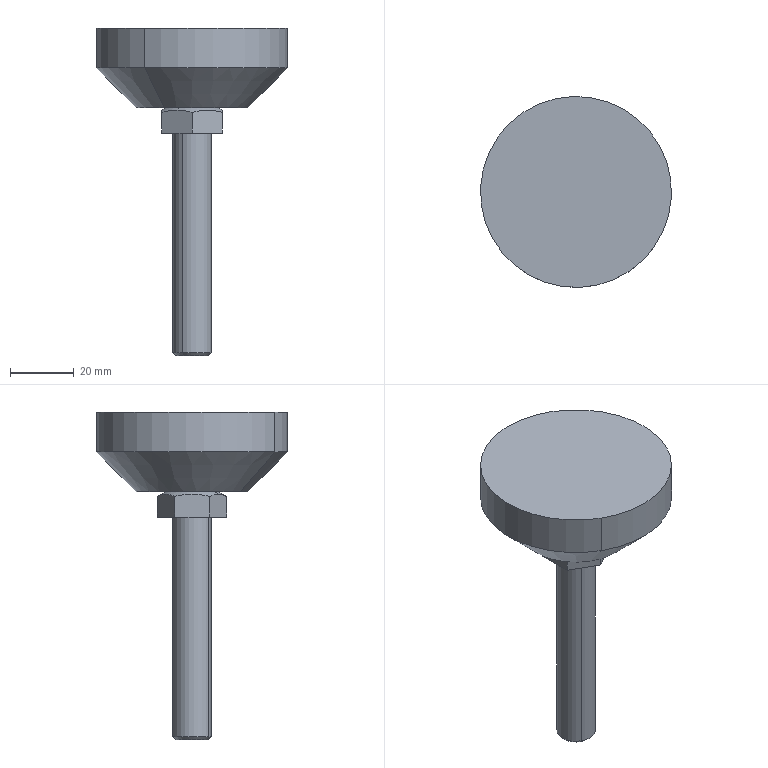Component | SolidWorks | FBR60_12_70-2_pad160_12_70pad1-1 | 1 solid | 25 faces | box 60 x 60 x 103 mm | volume 68306 mm3 | plane 11 | cylinder 8 | cone 6 | commonest cylinder face diameters 60 x2 27 x2 35 x2 12 x2
STEP:
#1=COLOUR_RGB('',0.7922,0.8196,0.9333);
#2=FILL_AREA_STYLE_COLOUR('',#1);
#3=FILL_AREA_STYLE('',(#2));
#4=SURFACE_STYLE_FILL_AREA(#3);
#5=SURFACE_SIDE_STYLE('',(#4));
#6=SURFACE_STYLE_USAGE(.BOTH.,#5);
#7=PRESENTATION_STYLE_ASSIGNMENT((#6));
#8=CARTESIAN_POINT('',(-32.646,-30.004,-16.848));
#9=VERTEX_POINT('',#8);
#10=CARTESIAN_POINT('',(-31.961,-28.808,-16.848));
#11=VERTEX_POINT('',#10);
#12=CARTESIAN_POINT('',(-32.303,-29.406,-16.848));
#13=DIRECTION('',(-0.,0.,-1.));
#14=DIRECTION('',(-0.4969,-0.8678,0.));
#15=AXIS2_PLACEMENT_3D('',#12,#13,#14);
#16=CIRCLE('',#15,0.689);
#17=EDGE_CURVE('',#9,#11,#16,.T.);
#18=ORIENTED_EDGE('',*,*,#17,.F.);
#19=CARTESIAN_POINT('',(-32.89,-30.431,-16.355));
#20=VERTEX_POINT('',#19);
#21=CARTESIAN_POINT('',(-32.89,-30.431,-16.355));
#22=DIRECTION('',(-0.3514,-0.6136,0.7071));
#23=VECTOR('',#22,39.37);
#24=LINE('',#21,#23);
#25=EDGE_CURVE('',#9,#20,#24,.T.);
#26=ORIENTED_EDGE('',*,*,#25,.T.);
#27=CARTESIAN_POINT('',(-31.716,-28.381,-16.355));
#28=VERTEX_POINT('',#27);
#29=CARTESIAN_POINT('',(-32.303,-29.406,-16.355));
#30=DIRECTION('',(-0.,0.,-1.));
#31=DIRECTION('',(-0.4969,-0.8678,0.));
#32=AXIS2_PLACEMENT_3D('',#29,#30,#31);
#33=CIRCLE('',#32,1.181);
#34=EDGE_CURVE('',#20,#28,#33,.T.);
#35=ORIENTED_EDGE('',*,*,#34,.T.);
#36=CARTESIAN_POINT('',(-31.716,-28.381,-16.355));
#37=DIRECTION('',(0.3514,0.6136,0.7071));
#38=VECTOR('',#37,39.37);
#39=LINE('',#36,#38);
#40=EDGE_CURVE('',#11,#28,#39,.T.);
#41=ORIENTED_EDGE('',*,*,#40,.F.);
#42=EDGE_LOOP('',(#18,#26,#35,#41));
#43=FACE_OUTER_BOUND('',#42,.T.);
#44=CARTESIAN_POINT('',(-32.303,-29.406,-16.355));
#45=DIRECTION('',(0.,-0.,1.));
#46=DIRECTION('',(0.4969,0.8678,0.));
#47=AXIS2_PLACEMENT_3D('',#44,#45,#46);
#48=CONICAL_SURFACE('',#47,1.181,0.7854);
#49=ADVANCED_FACE('',(#43),#48,.T.);
#50=CARTESIAN_POINT('',(-32.89,-30.431,-15.863));
#51=VERTEX_POINT('',#50);
#52=CARTESIAN_POINT('',(-31.716,-28.381,-15.863));
#53=VERTEX_POINT('',#52);
#54=CARTESIAN_POINT('',(-32.303,-29.406,-15.863));
#55=DIRECTION('',(-0.,0.,-1.));
#56=DIRECTION('',(-0.4969,-0.8678,0.));
#57=AXIS2_PLACEMENT_3D('',#54,#55,#56);
#58=CIRCLE('',#57,1.181);
#59=EDGE_CURVE('',#51,#53,#58,.T.);
#60=ORIENTED_EDGE('',*,*,#59,.T.);
#61=CARTESIAN_POINT('',(-31.716,-28.381,-15.863));
#62=DIRECTION('',(-0.,0.,-1.));
#63=VECTOR('',#62,39.37);
#64=LINE('',#61,#63);
#65=EDGE_CURVE('',#53,#28,#64,.T.);
#66=ORIENTED_EDGE('',*,*,#65,.T.);
#67=ORIENTED_EDGE('',*,*,#34,.F.);
#68=CARTESIAN_POINT('',(-32.89,-30.431,-15.863));
#69=DIRECTION('',(-0.,0.,-1.));
#70=VECTOR('',#69,39.37);
#71=LINE('',#68,#70);
#72=EDGE_CURVE('',#51,#20,#71,.T.);
#73=ORIENTED_EDGE('',*,*,#72,.F.);
#74=EDGE_LOOP('',(#60,#66,#67,#73));
#75=FACE_OUTER_BOUND('',#74,.T.);
#76=CARTESIAN_POINT('',(-32.303,-29.406,-15.863));
#77=DIRECTION('',(-0.,0.,-1.));
#78=DIRECTION('',(-0.4969,-0.8678,0.));
#79=AXIS2_PLACEMENT_3D('',#76,#77,#78);
#80=CYLINDRICAL_SURFACE('',#79,1.181);
#81=ADVANCED_FACE('',(#75),#80,.T.);
#82=CARTESIAN_POINT('',(-32.567,-29.867,-16.844));
#83=VERTEX_POINT('',#82);
#84=CARTESIAN_POINT('',(-32.039,-28.945,-16.844));
#85=VERTEX_POINT('',#84);
#86=CARTESIAN_POINT('',(-32.303,-29.406,-16.844));
#87=DIRECTION('',(-0.,0.,-1.));
#88=DIRECTION('',(-0.4969,-0.8678,0.));
#89=AXIS2_PLACEMENT_3D('',#86,#87,#88);
#90=CIRCLE('',#89,0.5315);
#91=EDGE_CURVE('',#83,#85,#90,.T.);
#92=ORIENTED_EDGE('',*,*,#91,.T.);
#93=CARTESIAN_POINT('',(-32.039,-28.945,-16.848));
#94=VERTEX_POINT('',#93);
#95=CARTESIAN_POINT('',(-32.039,-28.945,-16.844));
#96=DIRECTION('',(-0.,0.,-1.));
#97=VECTOR('',#96,39.37);
#98=LINE('',#95,#97);
#99=EDGE_CURVE('',#85,#94,#98,.T.);
#100=ORIENTED_EDGE('',*,*,#99,.T.);
#101=CARTESIAN_POINT('',(-32.567,-29.867,-16.848));
#102=VERTEX_POINT('',#101);
#103=CARTESIAN_POINT('',(-32.303,-29.406,-16.848));
#104=DIRECTION('',(-0.,0.,-1.));
#105=DIRECTION('',(-0.4969,-0.8678,0.));
#106=AXIS2_PLACEMENT_3D('',#103,#104,#105);
#107=CIRCLE('',#106,0.5315);
#108=EDGE_CURVE('',#102,#94,#107,.T.);
#109=ORIENTED_EDGE('',*,*,#108,.F.);
#110=CARTESIAN_POINT('',(-32.567,-29.867,-16.844));
#111=DIRECTION('',(-0.,0.,-1.));
#112=VECTOR('',#111,39.37);
#113=LINE('',#110,#112);
#114=EDGE_CURVE('',#83,#102,#113,.T.);
#115=ORIENTED_EDGE('',*,*,#114,.F.);
#116=EDGE_LOOP('',(#92,#100,#109,#115));
#117=FACE_OUTER_BOUND('',#116,.T.);
#118=CARTESIAN_POINT('',(-32.303,-29.406,-16.844));
#119=DIRECTION('',(-0.,0.,-1.));
#120=DIRECTION('',(-0.4969,-0.8678,0.));
#121=AXIS2_PLACEMENT_3D('',#118,#119,#120);
#122=CYLINDRICAL_SURFACE('',#121,0.5315);
#123=ADVANCED_FACE('',(#117),#122,.T.);
#124=CARTESIAN_POINT('',(-31.961,-28.808,-16.844));
#125=VERTEX_POINT('',#124);
#126=CARTESIAN_POINT('',(-32.646,-30.004,-16.844));
#127=VERTEX_POINT('',#126);
#128=CARTESIAN_POINT('',(-32.303,-29.406,-16.844));
#129=DIRECTION('',(-0.,0.,-1.));
#130=DIRECTION('',(-0.4969,-0.8678,0.));
#131=AXIS2_PLACEMENT_3D('',#128,#129,#130);
#132=CIRCLE('',#131,0.689);
#133=EDGE_CURVE('',#125,#127,#132,.T.);
#134=ORIENTED_EDGE('',*,*,#133,.F.);
#135=CARTESIAN_POINT('',(-31.961,-28.808,-16.844));
#136=DIRECTION('',(-0.,0.,-1.));
#137=VECTOR('',#136,39.37);
#138=LINE('',#135,#137);
#139=EDGE_CURVE('',#125,#11,#138,.T.);
#140=ORIENTED_EDGE('',*,*,#139,.T.);
#141=CARTESIAN_POINT('',(-32.303,-29.406,-16.848));
#142=DIRECTION('',(-0.,0.,-1.));
#143=DIRECTION('',(-0.4969,-0.8678,0.));
#144=AXIS2_PLACEMENT_3D('',#141,#142,#143);
#145=CIRCLE('',#144,0.689);
#146=EDGE_CURVE('',#11,#9,#145,.T.);
#147=ORIENTED_EDGE('',*,*,#146,.T.);
#148=CARTESIAN_POINT('',(-32.646,-30.004,-16.844));
#149=DIRECTION('',(-0.,0.,-1.));
#150=VECTOR('',#149,39.37);
#151=LINE('',#148,#150);
#152=EDGE_CURVE('',#127,#9,#151,.T.);
#153=ORIENTED_EDGE('',*,*,#152,.F.);
#154=EDGE_LOOP('',(#134,#140,#147,#153));
#155=FACE_OUTER_BOUND('',#154,.T.);
#156=CARTESIAN_POINT('',(-32.303,-29.406,-16.844));
#157=DIRECTION('',(-0.,0.,-1.));
#158=DIRECTION('',(-0.4969,-0.8678,0.));
#159=AXIS2_PLACEMENT_3D('',#156,#157,#158);
#160=CYLINDRICAL_SURFACE('',#159,0.689);
#161=ADVANCED_FACE('',(#155),#160,.F.);
#162=CARTESIAN_POINT('',(-32.421,-29.611,-17.163));
#163=VERTEX_POINT('',#162);
#164=CARTESIAN_POINT('',(-32.186,-29.201,-17.163));
#165=VERTEX_POINT('',#164);
#166=CARTESIAN_POINT('',(-32.303,-29.406,-17.163));
#167=DIRECTION('',(-0.,0.,-1.));
#168=DIRECTION('',(-0.4969,-0.8678,0.));
#169=AXIS2_PLACEMENT_3D('',#166,#167,#168);
#170=CIRCLE('',#169,0.2362);
#171=EDGE_CURVE('',#163,#165,#170,.T.);
#172=ORIENTED_EDGE('',*,*,#171,.T.);
#173=CARTESIAN_POINT('',(-32.186,-29.201,-19.881));
#174=VERTEX_POINT('',#173);
#175=CARTESIAN_POINT('',(-32.186,-29.201,-15.863));
#176=DIRECTION('',(-0.,0.,-1.));
#177=VECTOR('',#176,39.37);
#178=LINE('',#175,#177);
#179=EDGE_CURVE('',#165,#174,#178,.T.);
#180=ORIENTED_EDGE('',*,*,#179,.T.);
#181=CARTESIAN_POINT('',(-32.421,-29.611,-19.881));
#182=VERTEX_POINT('',#181);
#183=CARTESIAN_POINT('',(-32.303,-29.406,-19.881));
#184=DIRECTION('',(-0.,0.,-1.));
#185=DIRECTION('',(-0.4969,-0.8678,0.));
#186=AXIS2_PLACEMENT_3D('',#183,#184,#185);
#187=CIRCLE('',#186,0.2362);
#188=EDGE_CURVE('',#182,#174,#187,.T.);
#189=ORIENTED_EDGE('',*,*,#188,.F.);
#190=CARTESIAN_POINT('',(-32.421,-29.611,-15.863));
#191=DIRECTION('',(-0.,0.,-1.));
#192=VECTOR('',#191,39.37);
#193=LINE('',#190,#192);
#194=EDGE_CURVE('',#163,#182,#193,.T.);
#195=ORIENTED_EDGE('',*,*,#194,.F.);
#196=EDGE_LOOP('',(#172,#180,#189,#195));
#197=FACE_OUTER_BOUND('',#196,.T.);
#198=CARTESIAN_POINT('',(-32.303,-29.406,-15.863));
#199=DIRECTION('',(-0.,0.,-1.));
#200=DIRECTION('',(-0.4969,-0.8678,0.));
#201=AXIS2_PLACEMENT_3D('',#198,#199,#200);
#202=CYLINDRICAL_SURFACE('',#201,0.2362);
#203=ADVANCED_FACE('',(#197),#202,.T.);
#204=CARTESIAN_POINT('',(-32.402,-29.579,-19.918));
#205=VERTEX_POINT('',#204);
#206=CARTESIAN_POINT('',(-32.205,-29.233,-19.918));
#207=VERTEX_POINT('',#206);
#208=CARTESIAN_POINT('',(-32.303,-29.406,-19.918));
#209=DIRECTION('',(-0.,0.,-1.));
#210=DIRECTION('',(-0.4969,-0.8678,0.));
#211=AXIS2_PLACEMENT_3D('',#208,#209,#210);
#212=CIRCLE('',#211,0.1989);
#213=EDGE_CURVE('',#205,#207,#212,.T.);
#214=ORIENTED_EDGE('',*,*,#213,.F.);
#215=CARTESIAN_POINT('',(-32.421,-29.611,-19.881));
#216=DIRECTION('',(-0.3514,-0.6136,0.7071));
#217=VECTOR('',#216,39.37);
#218=LINE('',#215,#217);
#219=EDGE_CURVE('',#205,#182,#218,.T.);
#220=ORIENTED_EDGE('',*,*,#219,.T.);
#221=ORIENTED_EDGE('',*,*,#188,.T.);
#222=CARTESIAN_POINT('',(-32.186,-29.201,-19.881));
#223=DIRECTION('',(0.3514,0.6136,0.7071));
#224=VECTOR('',#223,39.37);
#225=LINE('',#222,#224);
#226=EDGE_CURVE('',#207,#174,#225,.T.);
#227=ORIENTED_EDGE('',*,*,#226,.F.);
#228=EDGE_LOOP('',(#214,#220,#221,#227));
#229=FACE_OUTER_BOUND('',#228,.T.);
#230=CARTESIAN_POINT('',(-32.303,-29.406,-19.881));
#231=DIRECTION('',(0.,-0.,1.));
#232=DIRECTION('',(0.4969,0.8678,0.));
#233=AXIS2_PLACEMENT_3D('',#230,#231,#232);
#234=CONICAL_SURFACE('',#233,0.2362,0.7854);
#235=ADVANCED_FACE('',(#229),#234,.T.);
#236=CARTESIAN_POINT('',(-32.46,-29.679,-16.848));
#237=VERTEX_POINT('',#236);
#238=CARTESIAN_POINT('',(-32.147,-29.133,-16.848));
#239=VERTEX_POINT('',#238);
#240=CARTESIAN_POINT('',(-32.303,-29.406,-16.848));
#241=DIRECTION('',(-0.,0.,-1.));
#242=DIRECTION('',(-0.4969,-0.8678,0.));
#243=AXIS2_PLACEMENT_3D('',#240,#241,#242);
#244=CIRCLE('',#243,0.315);
#245=EDGE_CURVE('',#237,#239,#244,.T.);
#246=ORIENTED_EDGE('',*,*,#245,.T.);
#247=CARTESIAN_POINT('',(-32.118,-29.081,-16.878));
#248=VERTEX_POINT('',#247);
#249=CARTESIAN_POINT('',(-32.147,-29.133,-16.848));
#250=DIRECTION('',(0.4416,0.7711,-0.4586));
#251=VECTOR('',#250,39.37);
#252=LINE('',#249,#251);
#253=EDGE_CURVE('',#239,#248,#252,.T.);
#254=ORIENTED_EDGE('',*,*,#253,.T.);
#255=CARTESIAN_POINT('',(-32.305,-28.974,-16.908));
#256=VERTEX_POINT('',#255);
#257=CARTESIAN_POINT('',(-32.118,-29.081,-16.878));
#258=CARTESIAN_POINT('',(-32.149,-29.063,-16.878));
#259=CARTESIAN_POINT('',(-32.181,-29.045,-16.881));
#260=CARTESIAN_POINT('',(-32.244,-29.009,-16.891));
#261=CARTESIAN_POINT('',(-32.274,-28.992,-16.899));
#262=CARTESIAN_POINT('',(-32.305,-28.974,-16.908));
#263=B_SPLINE_CURVE_WITH_KNOTS('',3,(#257,#258,#259,#260,#261,#262),.UNSPECIFIED.,.F.,.F.,(4,2,4),(0.01513,0.01791,0.02068),.UNSPECIFIED.);
#264=EDGE_CURVE('',#248,#256,#263,.T.);
#265=ORIENTED_EDGE('',*,*,#264,.T.);
#266=CARTESIAN_POINT('',(-32.678,-29.191,-16.908));
#267=VERTEX_POINT('',#266);
#268=CARTESIAN_POINT('',(-32.305,-28.974,-16.908));
#269=CARTESIAN_POINT('',(-32.336,-28.992,-16.899));
#270=CARTESIAN_POINT('',(-32.366,-29.01,-16.891));
#271=CARTESIAN_POINT('',(-32.428,-29.046,-16.881));
#272=CARTESIAN_POINT('',(-32.459,-29.064,-16.878));
#273=CARTESIAN_POINT('',(-32.506,-29.091,-16.878));
#274=CARTESIAN_POINT('',(-32.522,-29.101,-16.879));
#275=CARTESIAN_POINT('',(-32.554,-29.119,-16.881));
#276=CARTESIAN_POINT('',(-32.569,-29.128,-16.883));
#277=CARTESIAN_POINT('',(-32.616,-29.155,-16.891));
#278=CARTESIAN_POINT('',(-32.647,-29.174,-16.899));
#279=CARTESIAN_POINT('',(-32.678,-29.191,-16.908));
#280=B_SPLINE_CURVE_WITH_KNOTS('',3,(#268,#269,#270,#271,#272,#273,#274,#275,#276,#277,#278,#279),.UNSPECIFIED.,.F.,.F.,(4,2,2,2,2,4),(0.00000024,0.002752,0.005505,0.006881,0.008257,0.01101),.UNSPECIFIED.);
#281=EDGE_CURVE('',#256,#267,#280,.T.);
#282=ORIENTED_EDGE('',*,*,#281,.T.);
#283=CARTESIAN_POINT('',(-32.677,-29.623,-16.908));
#284=VERTEX_POINT('',#283);
#285=CARTESIAN_POINT('',(-32.678,-29.191,-16.908));
#286=CARTESIAN_POINT('',(-32.678,-29.227,-16.899));
#287=CARTESIAN_POINT('',(-32.678,-29.262,-16.891));
#288=CARTESIAN_POINT('',(-32.678,-29.334,-16.881));
#289=CARTESIAN_POINT('',(-32.678,-29.37,-16.878));
#290=CARTESIAN_POINT('',(-32.677,-29.424,-16.878));
#291=CARTESIAN_POINT('',(-32.677,-29.443,-16.879));
#292=CARTESIAN_POINT('',(-32.677,-29.479,-16.881));
#293=CARTESIAN_POINT('',(-32.677,-29.497,-16.883));
#294=CARTESIAN_POINT('',(-32.677,-29.552,-16.891));
#295=CARTESIAN_POINT('',(-32.677,-29.588,-16.899));
#296=CARTESIAN_POINT('',(-32.677,-29.623,-16.908));
#297=B_SPLINE_CURVE_WITH_KNOTS('',3,(#285,#286,#287,#288,#289,#290,#291,#292,#293,#294,#295,#296),.UNSPECIFIED.,.F.,.F.,(4,2,2,2,2,4),(0.00000024,0.002752,0.005505,0.006881,0.008257,0.01101),.UNSPECIFIED.);
#298=EDGE_CURVE('',#267,#284,#297,.T.);
#299=ORIENTED_EDGE('',*,*,#298,.T.);
#300=CARTESIAN_POINT('',(-32.489,-29.731,-16.878));
#301=VERTEX_POINT('',#300);
#302=CARTESIAN_POINT('',(-32.677,-29.623,-16.908));
#303=CARTESIAN_POINT('',(-32.646,-29.641,-16.899));
#304=CARTESIAN_POINT('',(-32.615,-29.658,-16.891));
#305=CARTESIAN_POINT('',(-32.553,-29.694,-16.881));
#306=CARTESIAN_POINT('',(-32.521,-29.712,-16.878));
#307=CARTESIAN_POINT('',(-32.489,-29.731,-16.878));
#308=B_SPLINE_CURVE_WITH_KNOTS('',3,(#302,#303,#304,#305,#306,#307),.UNSPECIFIED.,.F.,.F.,(4,2,4),(0.00514,0.007899,0.01066),.UNSPECIFIED.);
#309=EDGE_CURVE('',#284,#301,#308,.T.);
#310=ORIENTED_EDGE('',*,*,#309,.T.);
#311=CARTESIAN_POINT('',(-32.46,-29.679,-16.848));
#312=DIRECTION('',(-0.4416,-0.7711,-0.4586));
#313=VECTOR('',#312,39.37);
#314=LINE('',#311,#313);
#315=EDGE_CURVE('',#237,#301,#314,.T.);
#316=ORIENTED_EDGE('',*,*,#315,.F.);
#317=EDGE_LOOP('',(#246,#254,#265,#282,#299,#310,#316));
#318=FACE_OUTER_BOUND('',#317,.T.);
#319=CARTESIAN_POINT('',(-32.303,-29.406,-16.848));
#320=DIRECTION('',(-0.,0.,-1.));
#321=DIRECTION('',(-0.4969,-0.8678,0.));
#322=AXIS2_PLACEMENT_3D('',#319,#320,#321);
#323=CONICAL_SURFACE('',#322,0.315,1.094);
#324=ADVANCED_FACE('',(#318),#323,.T.);
#325=ORIENTED_EDGE('',*,*,#245,.F.);
#326=CARTESIAN_POINT('',(-32.303,-29.406,-16.848));
#327=DIRECTION('',(-0.,0.,-1.));
#328=DIRECTION('',(-0.4969,-0.8678,0.));
#329=AXIS2_PLACEMENT_3D('',#326,#327,#328);
#330=CIRCLE('',#329,0.315);
#331=EDGE_CURVE('',#239,#237,#330,.T.);
#332=ORIENTED_EDGE('',*,*,#331,.F.);
#333=EDGE_LOOP('',(#325,#332));
#334=FACE_BOUND('',#333,.T.);
#335=ORIENTED_EDGE('',*,*,#108,.T.);
#336=CARTESIAN_POINT('',(-32.303,-29.406,-16.848));
#337=DIRECTION('',(-0.,0.,-1.));
#338=DIRECTION('',(-0.4969,-0.8678,0.));
#339=AXIS2_PLACEMENT_3D('',#336,#337,#338);
#340=CIRCLE('',#339,0.5315);
#341=EDGE_CURVE('',#94,#102,#340,.T.);
#342=ORIENTED_EDGE('',*,*,#341,.T.);
#343=EDGE_LOOP('',(#335,#342));
#344=FACE_OUTER_BOUND('',#343,.T.);
#345=CARTESIAN_POINT('',(-32.577,-29.25,-16.848));
#346=DIRECTION('',(0.,-0.,1.));
#347=DIRECTION('',(0.4969,0.8678,0.));
#348=AXIS2_PLACEMENT_3D('',#345,#346,#347);
#349=PLANE('',#348);
#350=ADVANCED_FACE('',(#334,#344),#349,.F.);
#351=ORIENTED_EDGE('',*,*,#253,.F.);
#352=ORIENTED_EDGE('',*,*,#331,.T.);
#353=ORIENTED_EDGE('',*,*,#315,.T.);
#354=CARTESIAN_POINT('',(-32.302,-29.838,-16.908));
#355=VERTEX_POINT('',#354);
#356=CARTESIAN_POINT('',(-32.489,-29.731,-16.878));
#357=CARTESIAN_POINT('',(-32.458,-29.749,-16.878));
#358=CARTESIAN_POINT('',(-32.426,-29.767,-16.881));
#359=CARTESIAN_POINT('',(-32.364,-29.802,-16.891));
#360=CARTESIAN_POINT('',(-32.332,-29.82,-16.899));
#361=CARTESIAN_POINT('',(-32.302,-29.838,-16.908));
#362=B_SPLINE_CURVE_WITH_KNOTS('',3,(#356,#357,#358,#359,#360,#361),.UNSPECIFIED.,.F.,.F.,(4,2,4),(0.01066,0.01341,0.01617),.UNSPECIFIED.);
#363=EDGE_CURVE('',#301,#355,#362,.T.);
#364=ORIENTED_EDGE('',*,*,#363,.T.);
#365=CARTESIAN_POINT('',(-31.929,-29.621,-16.908));
#366=VERTEX_POINT('',#365);
#367=CARTESIAN_POINT('',(-32.302,-29.838,-16.908));
#368=CARTESIAN_POINT('',(-32.271,-29.82,-16.899));
#369=CARTESIAN_POINT('',(-32.24,-29.802,-16.891));
#370=CARTESIAN_POINT('',(-32.179,-29.766,-16.881));
#371=CARTESIAN_POINT('',(-32.147,-29.748,-16.878));
#372=CARTESIAN_POINT('',(-32.1,-29.721,-16.878));
#373=CARTESIAN_POINT('',(-32.085,-29.712,-16.879));
#374=CARTESIAN_POINT('',(-32.053,-29.693,-16.881));
#375=CARTESIAN_POINT('',(-32.037,-29.684,-16.883));
#376=CARTESIAN_POINT('',(-31.99,-29.657,-16.891));
#377=CARTESIAN_POINT('',(-31.959,-29.639,-16.899));
#378=CARTESIAN_POINT('',(-31.929,-29.621,-16.908));
#379=B_SPLINE_CURVE_WITH_KNOTS('',3,(#367,#368,#369,#370,#371,#372,#373,#374,#375,#376,#377,#378),.UNSPECIFIED.,.F.,.F.,(4,2,2,2,2,4),(0.00000024,0.002752,0.005505,0.006881,0.008257,0.01101),.UNSPECIFIED.);
#380=EDGE_CURVE('',#355,#366,#379,.T.);
#381=ORIENTED_EDGE('',*,*,#380,.T.);
#382=CARTESIAN_POINT('',(-31.93,-29.189,-16.908));
#383=VERTEX_POINT('',#382);
#384=CARTESIAN_POINT('',(-31.929,-29.621,-16.908));
#385=CARTESIAN_POINT('',(-31.929,-29.585,-16.899));
#386=CARTESIAN_POINT('',(-31.929,-29.55,-16.891));
#387=CARTESIAN_POINT('',(-31.929,-29.478,-16.881));
#388=CARTESIAN_POINT('',(-31.929,-29.442,-16.878));
#389=CARTESIAN_POINT('',(-31.929,-29.388,-16.878));
#390=CARTESIAN_POINT('',(-31.929,-29.369,-16.879));
#391=CARTESIAN_POINT('',(-31.93,-29.333,-16.881));
#392=CARTESIAN_POINT('',(-31.93,-29.315,-16.883));
#393=CARTESIAN_POINT('',(-31.93,-29.26,-16.891));
#394=CARTESIAN_POINT('',(-31.93,-29.224,-16.899));
#395=CARTESIAN_POINT('',(-31.93,-29.189,-16.908));
#396=B_SPLINE_CURVE_WITH_KNOTS('',3,(#384,#385,#386,#387,#388,#389,#390,#391,#392,#393,#394,#395),.UNSPECIFIED.,.F.,.F.,(4,2,2,2,2,4),(0.00000024,0.002752,0.005505,0.006881,0.008257,0.01101),.UNSPECIFIED.);
#397=EDGE_CURVE('',#366,#383,#396,.T.);
#398=ORIENTED_EDGE('',*,*,#397,.T.);
#399=CARTESIAN_POINT('',(-31.93,-29.189,-16.908));
#400=CARTESIAN_POINT('',(-31.961,-29.171,-16.899));
#401=CARTESIAN_POINT('',(-31.992,-29.153,-16.891));
#402=CARTESIAN_POINT('',(-32.055,-29.118,-16.881));
#403=CARTESIAN_POINT('',(-32.086,-29.1,-16.878));
#404=CARTESIAN_POINT('',(-32.118,-29.081,-16.878));
#405=B_SPLINE_CURVE_WITH_KNOTS('',3,(#399,#400,#401,#402,#403,#404),.UNSPECIFIED.,.F.,.F.,(4,2,4),(0.0096,0.01237,0.01513),.UNSPECIFIED.);
#406=EDGE_CURVE('',#383,#248,#405,.T.);
#407=ORIENTED_EDGE('',*,*,#406,.T.);
#408=EDGE_LOOP('',(#351,#352,#353,#364,#381,#398,#407));
#409=FACE_OUTER_BOUND('',#408,.T.);
#410=CARTESIAN_POINT('',(-32.303,-29.406,-16.848));
#411=DIRECTION('',(-0.,0.,-1.));
#412=DIRECTION('',(-0.4969,-0.8678,0.));
#413=AXIS2_PLACEMENT_3D('',#410,#411,#412);
#414=CONICAL_SURFACE('',#413,0.315,1.094);
#415=ADVANCED_FACE('',(#409),#414,.T.);
#416=CARTESIAN_POINT('',(-31.93,-29.189,-17.163));
#417=VERTEX_POINT('',#416);
#418=CARTESIAN_POINT('',(-31.93,-29.189,-17.202));
#419=DIRECTION('',(0.,-0.,1.));
#420=VECTOR('',#419,39.37);
#421=LINE('',#418,#420);
#422=EDGE_CURVE('',#417,#383,#421,.T.);
#423=ORIENTED_EDGE('',*,*,#422,.T.);
#424=ORIENTED_EDGE('',*,*,#397,.F.);
#425=CARTESIAN_POINT('',(-31.929,-29.621,-17.163));
#426=VERTEX_POINT('',#425);
#427=CARTESIAN_POINT('',(-31.929,-29.621,-17.202));
#428=DIRECTION('',(0.,-0.,1.));
#429=VECTOR('',#428,39.37);
#430=LINE('',#427,#429);
#431=EDGE_CURVE('',#426,#366,#430,.T.);
#432=ORIENTED_EDGE('',*,*,#431,.F.);
#433=CARTESIAN_POINT('',(-31.93,-29.287,-17.163));
#434=DIRECTION('',(0.003538,-1.,-0.));
#435=VECTOR('',#434,39.37);
#436=LINE('',#433,#435);
#437=EDGE_CURVE('',#417,#426,#436,.T.);
#438=ORIENTED_EDGE('',*,*,#437,.F.);
#439=EDGE_LOOP('',(#423,#424,#432,#438));
#440=FACE_OUTER_BOUND('',#439,.T.);
#441=CARTESIAN_POINT('',(-31.93,-29.189,-17.202));
#442=DIRECTION('',(-1.,-0.003538,0.));
#443=DIRECTION('',(-0.003538,1.,0.));
#444=AXIS2_PLACEMENT_3D('',#441,#442,#443);
#445=PLANE('',#444);
#446=ADVANCED_FACE('',(#440),#445,.F.);
#447=ORIENTED_EDGE('',*,*,#431,.T.);
#448=ORIENTED_EDGE('',*,*,#380,.F.);
#449=CARTESIAN_POINT('',(-32.302,-29.838,-17.163));
#450=VERTEX_POINT('',#449);
#451=CARTESIAN_POINT('',(-32.302,-29.838,-17.202));
#452=DIRECTION('',(0.,-0.,1.));
#453=VECTOR('',#452,39.37);
#454=LINE('',#451,#453);
#455=EDGE_CURVE('',#450,#355,#454,.T.);
#456=ORIENTED_EDGE('',*,*,#455,.F.);
#457=CARTESIAN_POINT('',(-32.217,-29.789,-17.163));
#458=DIRECTION('',(-0.8643,-0.5031,-0.));
#459=VECTOR('',#458,39.37);
#460=LINE('',#457,#459);
#461=EDGE_CURVE('',#426,#450,#460,.T.);
#462=ORIENTED_EDGE('',*,*,#461,.F.);
#463=EDGE_LOOP('',(#447,#448,#456,#462));
#464=FACE_OUTER_BOUND('',#463,.T.);
#465=CARTESIAN_POINT('',(-31.929,-29.621,-17.202));
#466=DIRECTION('',(-0.5031,0.8643,0.));
#467=DIRECTION('',(0.8643,0.5031,0.));
#468=AXIS2_PLACEMENT_3D('',#465,#466,#467);
#469=PLANE('',#468);
#470=ADVANCED_FACE('',(#464),#469,.F.);
#471=ORIENTED_EDGE('',*,*,#455,.T.);
#472=ORIENTED_EDGE('',*,*,#363,.F.);
#473=ORIENTED_EDGE('',*,*,#309,.F.);
#474=CARTESIAN_POINT('',(-32.677,-29.623,-17.163));
#475=VERTEX_POINT('',#474);
#476=CARTESIAN_POINT('',(-32.677,-29.623,-17.202));
#477=DIRECTION('',(0.,-0.,1.));
#478=VECTOR('',#477,39.37);
#479=LINE('',#476,#478);
#480=EDGE_CURVE('',#475,#284,#479,.T.);
#481=ORIENTED_EDGE('',*,*,#480,.F.);
#482=CARTESIAN_POINT('',(-32.694,-29.613,-17.163));
#483=DIRECTION('',(-0.8678,0.4969,0.));
#484=VECTOR('',#483,39.37);
#485=LINE('',#482,#484);
#486=EDGE_CURVE('',#450,#475,#485,.T.);
#487=ORIENTED_EDGE('',*,*,#486,.F.);
#488=EDGE_LOOP('',(#471,#472,#473,#481,#487));
#489=FACE_OUTER_BOUND('',#488,.T.);
#490=CARTESIAN_POINT('',(-32.302,-29.838,-17.202));
#491=DIRECTION('',(0.4969,0.8678,0.));
#492=DIRECTION('',(0.8678,-0.4969,-0.));
#493=AXIS2_PLACEMENT_3D('',#490,#491,#492);
#494=PLANE('',#493);
#495=ADVANCED_FACE('',(#489),#494,.F.);
#496=ORIENTED_EDGE('',*,*,#480,.T.);
#497=ORIENTED_EDGE('',*,*,#298,.F.);
#498=CARTESIAN_POINT('',(-32.678,-29.191,-17.163));
#499=VERTEX_POINT('',#498);
#500=CARTESIAN_POINT('',(-32.678,-29.191,-17.202));
#501=DIRECTION('',(0.,-0.,1.));
#502=VECTOR('',#501,39.37);
#503=LINE('',#500,#502);
#504=EDGE_CURVE('',#499,#267,#503,.T.);
#505=ORIENTED_EDGE('',*,*,#504,.F.);
#506=CARTESIAN_POINT('',(-32.678,-29.289,-17.163));
#507=DIRECTION('',(-0.003538,1.,0.));
#508=VECTOR('',#507,39.37);
#509=LINE('',#506,#508);
#510=EDGE_CURVE('',#475,#499,#509,.T.);
#511=ORIENTED_EDGE('',*,*,#510,.F.);
#512=EDGE_LOOP('',(#496,#497,#505,#511));
#513=FACE_OUTER_BOUND('',#512,.T.);
#514=CARTESIAN_POINT('',(-32.677,-29.623,-17.202));
#515=DIRECTION('',(1.,0.003538,-0.));
#516=DIRECTION('',(0.003538,-1.,-0.));
#517=AXIS2_PLACEMENT_3D('',#514,#515,#516);
#518=PLANE('',#517);
#519=ADVANCED_FACE('',(#513),#518,.F.);
#520=ORIENTED_EDGE('',*,*,#504,.T.);
#521=ORIENTED_EDGE('',*,*,#281,.F.);
#522=CARTESIAN_POINT('',(-32.305,-28.974,-17.163));
#523=VERTEX_POINT('',#522);
#524=CARTESIAN_POINT('',(-32.305,-28.974,-17.202));
#525=DIRECTION('',(0.,-0.,1.));
#526=VECTOR('',#525,39.37);
#527=LINE('',#524,#526);
#528=EDGE_CURVE('',#523,#256,#527,.T.);
#529=ORIENTED_EDGE('',*,*,#528,.F.);
#530=CARTESIAN_POINT('',(-32.594,-29.142,-17.163));
#531=DIRECTION('',(0.8643,0.5031,0.));
#532=VECTOR('',#531,39.37);
#533=LINE('',#530,#532);
#534=EDGE_CURVE('',#499,#523,#533,.T.);
#535=ORIENTED_EDGE('',*,*,#534,.F.);
#536=EDGE_LOOP('',(#520,#521,#529,#535));
#537=FACE_OUTER_BOUND('',#536,.T.);
#538=CARTESIAN_POINT('',(-32.678,-29.191,-17.202));
#539=DIRECTION('',(0.5031,-0.8643,-0.));
#540=DIRECTION('',(-0.8643,-0.5031,-0.));
#541=AXIS2_PLACEMENT_3D('',#538,#539,#540);
#542=PLANE('',#541);
#543=ADVANCED_FACE('',(#537),#542,.F.);
#544=ORIENTED_EDGE('',*,*,#528,.T.);
#545=ORIENTED_EDGE('',*,*,#264,.F.);
#546=ORIENTED_EDGE('',*,*,#406,.F.);
#547=ORIENTED_EDGE('',*,*,#422,.F.);
#548=CARTESIAN_POINT('',(-32.322,-28.964,-17.163));
#549=DIRECTION('',(0.8678,-0.4969,-0.));
#550=VECTOR('',#549,39.37);
#551=LINE('',#548,#550);
#552=EDGE_CURVE('',#523,#417,#551,.T.);
#553=ORIENTED_EDGE('',*,*,#552,.F.);
#554=EDGE_LOOP('',(#544,#545,#546,#547,#553));
#555=FACE_OUTER_BOUND('',#554,.T.);
#556=CARTESIAN_POINT('',(-32.305,-28.974,-17.202));
#557=DIRECTION('',(-0.4969,-0.8678,-0.));
#558=DIRECTION('',(-0.8678,0.4969,0.));
#559=AXIS2_PLACEMENT_3D('',#556,#557,#558);
#560=PLANE('',#559);
#561=ADVANCED_FACE('',(#555),#560,.F.);
#562=CARTESIAN_POINT('',(-32.303,-29.406,-19.918));
#563=DIRECTION('',(-0.,0.,-1.));
#564=DIRECTION('',(-0.4969,-0.8678,0.));
#565=AXIS2_PLACEMENT_3D('',#562,#563,#564);
#566=CIRCLE('',#565,0.1989);
#567=EDGE_CURVE('',#207,#205,#566,.T.);
#568=ORIENTED_EDGE('',*,*,#567,.T.);
#569=ORIENTED_EDGE('',*,*,#213,.T.);
#570=EDGE_LOOP('',(#568,#569));
#571=FACE_OUTER_BOUND('',#570,.T.);
#572=CARTESIAN_POINT('',(-32.303,-29.406,-19.918));
#573=DIRECTION('',(0.,-0.,1.));
#574=DIRECTION('',(0.4969,0.8678,0.));
#575=AXIS2_PLACEMENT_3D('',#572,#573,#574);
#576=PLANE('',#575);
#577=ADVANCED_FACE('',(#571),#576,.F.);
#578=ORIENTED_EDGE('',*,*,#219,.F.);
#579=ORIENTED_EDGE('',*,*,#567,.F.);
#580=ORIENTED_EDGE('',*,*,#226,.T.);
#581=CARTESIAN_POINT('',(-32.303,-29.406,-19.881));
#582=DIRECTION('',(-0.,0.,-1.));
#583=DIRECTION('',(-0.4969,-0.8678,0.));
#584=AXIS2_PLACEMENT_3D('',#581,#582,#583);
#585=CIRCLE('',#584,0.2362);
#586=EDGE_CURVE('',#174,#182,#585,.T.);
#587=ORIENTED_EDGE('',*,*,#586,.T.);
#588=EDGE_LOOP('',(#578,#579,#580,#587));
#589=FACE_OUTER_BOUND('',#588,.T.);
#590=CARTESIAN_POINT('',(-32.303,-29.406,-19.881));
#591=DIRECTION('',(0.,-0.,1.));
#592=DIRECTION('',(0.4969,0.8678,0.));
#593=AXIS2_PLACEMENT_3D('',#590,#591,#592);
#594=CONICAL_SURFACE('',#593,0.2362,0.7854);
#595=ADVANCED_FACE('',(#589),#594,.T.);
#596=ORIENTED_EDGE('',*,*,#179,.F.);
#597=CARTESIAN_POINT('',(-32.303,-29.406,-17.163));
#598=DIRECTION('',(-0.,0.,-1.));
#599=DIRECTION('',(-0.4969,-0.8678,0.));
#600=AXIS2_PLACEMENT_3D('',#597,#598,#599);
#601=CIRCLE('',#600,0.2362);
#602=EDGE_CURVE('',#165,#163,#601,.T.);
#603=ORIENTED_EDGE('',*,*,#602,.T.);
#604=ORIENTED_EDGE('',*,*,#194,.T.);
#605=ORIENTED_EDGE('',*,*,#586,.F.);
#606=EDGE_LOOP('',(#596,#603,#604,#605));
#607=FACE_OUTER_BOUND('',#606,.T.);
#608=CARTESIAN_POINT('',(-32.303,-29.406,-15.863));
#609=DIRECTION('',(-0.,0.,-1.));
#610=DIRECTION('',(-0.4969,-0.8678,0.));
#611=AXIS2_PLACEMENT_3D('',#608,#609,#610);
#612=CYLINDRICAL_SURFACE('',#611,0.2362);
#613=ADVANCED_FACE('',(#607),#612,.T.);
#614=ORIENTED_EDGE('',*,*,#552,.T.);
#615=ORIENTED_EDGE('',*,*,#437,.T.);
#616=ORIENTED_EDGE('',*,*,#461,.T.);
#617=ORIENTED_EDGE('',*,*,#486,.T.);
#618=ORIENTED_EDGE('',*,*,#510,.T.);
#619=ORIENTED_EDGE('',*,*,#534,.T.);
#620=EDGE_LOOP('',(#614,#615,#616,#617,#618,#619));
#621=FACE_OUTER_BOUND('',#620,.T.);
#622=ORIENTED_EDGE('',*,*,#171,.F.);
#623=ORIENTED_EDGE('',*,*,#602,.F.);
#624=EDGE_LOOP('',(#622,#623));
#625=FACE_BOUND('',#624,.T.);
#626=CARTESIAN_POINT('',(-32.508,-29.289,-17.163));
#627=DIRECTION('',(0.,-0.,1.));
#628=DIRECTION('',(0.4969,0.8678,0.));
#629=AXIS2_PLACEMENT_3D('',#626,#627,#628);
#630=PLANE('',#629);
#631=ADVANCED_FACE('',(#621,#625),#630,.F.);
#632=ORIENTED_EDGE('',*,*,#139,.F.);
#633=CARTESIAN_POINT('',(-32.303,-29.406,-16.844));
#634=DIRECTION('',(-0.,0.,-1.));
#635=DIRECTION('',(-0.4969,-0.8678,0.));
#636=AXIS2_PLACEMENT_3D('',#633,#634,#635);
#637=CIRCLE('',#636,0.689);
#638=EDGE_CURVE('',#127,#125,#637,.T.);
#639=ORIENTED_EDGE('',*,*,#638,.F.);
#640=ORIENTED_EDGE('',*,*,#152,.T.);
#641=ORIENTED_EDGE('',*,*,#17,.T.);
#642=EDGE_LOOP('',(#632,#639,#640,#641));
#643=FACE_OUTER_BOUND('',#642,.T.);
#644=CARTESIAN_POINT('',(-32.303,-29.406,-16.844));
#645=DIRECTION('',(-0.,0.,-1.));
#646=DIRECTION('',(-0.4969,-0.8678,0.));
#647=AXIS2_PLACEMENT_3D('',#644,#645,#646);
#648=CYLINDRICAL_SURFACE('',#647,0.689);
#649=ADVANCED_FACE('',(#643),#648,.F.);
#650=ORIENTED_EDGE('',*,*,#91,.F.);
#651=CARTESIAN_POINT('',(-32.303,-29.406,-16.844));
#652=DIRECTION('',(-0.,0.,-1.));
#653=DIRECTION('',(-0.4969,-0.8678,0.));
#654=AXIS2_PLACEMENT_3D('',#651,#652,#653);
#655=CIRCLE('',#654,0.5315);
#656=EDGE_CURVE('',#85,#83,#655,.T.);
#657=ORIENTED_EDGE('',*,*,#656,.F.);
#658=EDGE_LOOP('',(#650,#657));
#659=FACE_BOUND('',#658,.T.);
#660=ORIENTED_EDGE('',*,*,#638,.T.);
#661=ORIENTED_EDGE('',*,*,#133,.T.);
#662=EDGE_LOOP('',(#660,#661));
#663=FACE_OUTER_BOUND('',#662,.T.);
#664=CARTESIAN_POINT('',(-32.303,-29.406,-16.844));
#665=DIRECTION('',(-0.,0.,-1.));
#666=DIRECTION('',(-0.4969,-0.8678,-0.));
#667=AXIS2_PLACEMENT_3D('',#664,#665,#666);
#668=PLANE('',#667);
#669=ADVANCED_FACE('',(#659,#663),#668,.T.);
#670=ORIENTED_EDGE('',*,*,#99,.F.);
#671=ORIENTED_EDGE('',*,*,#656,.T.);
#672=ORIENTED_EDGE('',*,*,#114,.T.);
#673=ORIENTED_EDGE('',*,*,#341,.F.);
#674=EDGE_LOOP('',(#670,#671,#672,#673));
#675=FACE_OUTER_BOUND('',#674,.T.);
#676=CARTESIAN_POINT('',(-32.303,-29.406,-16.844));
#677=DIRECTION('',(-0.,0.,-1.));
#678=DIRECTION('',(-0.4969,-0.8678,0.));
#679=AXIS2_PLACEMENT_3D('',#676,#677,#678);
#680=CYLINDRICAL_SURFACE('',#679,0.5315);
#681=ADVANCED_FACE('',(#675),#680,.T.);
#682=ORIENTED_EDGE('',*,*,#59,.F.);
#683=CARTESIAN_POINT('',(-32.303,-29.406,-15.863));
#684=DIRECTION('',(-0.,0.,-1.));
#685=DIRECTION('',(-0.4969,-0.8678,0.));
#686=AXIS2_PLACEMENT_3D('',#683,#684,#685);
#687=CIRCLE('',#686,1.181);
#688=EDGE_CURVE('',#53,#51,#687,.T.);
#689=ORIENTED_EDGE('',*,*,#688,.F.);
#690=EDGE_LOOP('',(#682,#689));
#691=FACE_OUTER_BOUND('',#690,.T.);
#692=CARTESIAN_POINT('',(-33.328,-28.819,-15.863));
#693=DIRECTION('',(-0.,0.,-1.));
#694=DIRECTION('',(-0.4969,-0.8678,-0.));
#695=AXIS2_PLACEMENT_3D('',#692,#693,#694);
#696=PLANE('',#695);
#697=ADVANCED_FACE('',(#691),#696,.F.);
#698=ORIENTED_EDGE('',*,*,#65,.F.);
#699=ORIENTED_EDGE('',*,*,#688,.T.);
#700=ORIENTED_EDGE('',*,*,#72,.T.);
#701=CARTESIAN_POINT('',(-32.303,-29.406,-16.355));
#702=DIRECTION('',(-0.,0.,-1.));
#703=DIRECTION('',(-0.4969,-0.8678,0.));
#704=AXIS2_PLACEMENT_3D('',#701,#702,#703);
#705=CIRCLE('',#704,1.181);
#706=EDGE_CURVE('',#28,#20,#705,.T.);
#707=ORIENTED_EDGE('',*,*,#706,.F.);
#708=EDGE_LOOP('',(#698,#699,#700,#707));
#709=FACE_OUTER_BOUND('',#708,.T.);
#710=CARTESIAN_POINT('',(-32.303,-29.406,-15.863));
#711=DIRECTION('',(-0.,0.,-1.));
#712=DIRECTION('',(-0.4969,-0.8678,0.));
#713=AXIS2_PLACEMENT_3D('',#710,#711,#712);
#714=CYLINDRICAL_SURFACE('',#713,1.181);
#715=ADVANCED_FACE('',(#709),#714,.T.);
#716=ORIENTED_EDGE('',*,*,#25,.F.);
#717=ORIENTED_EDGE('',*,*,#146,.F.);
#718=ORIENTED_EDGE('',*,*,#40,.T.);
#719=ORIENTED_EDGE('',*,*,#706,.T.);
#720=EDGE_LOOP('',(#716,#717,#718,#719));
#721=FACE_OUTER_BOUND('',#720,.T.);
#722=CARTESIAN_POINT('',(-32.303,-29.406,-16.355));
#723=DIRECTION('',(0.,-0.,1.));
#724=DIRECTION('',(0.4969,0.8678,0.));
#725=AXIS2_PLACEMENT_3D('',#722,#723,#724);
#726=CONICAL_SURFACE('',#725,1.181,0.7854);
#727=ADVANCED_FACE('',(#721),#726,.T.);
#728=CLOSED_SHELL('',(#49,#81,#123,#161,#203,#235,#324,#350,#415,#446,#470,#495,#519,#543,#561,#577,#595,#613,#631,#649,#669,#681,#697,#715,#727));
#729=MANIFOLD_SOLID_BREP('',#728);
#730=STYLED_ITEM('',(#7),#729);
#731=(LENGTH_UNIT()NAMED_UNIT(*)SI_UNIT($,.METRE.));
#732=LENGTH_MEASURE_WITH_UNIT(LENGTH_MEASURE(0.0254),#731);
#733=DIMENSIONAL_EXPONENTS(1.,0.,0.,0.,0.,0.,0.);
#734=(CONVERSION_BASED_UNIT('',#732)LENGTH_UNIT()NAMED_UNIT(#733));
#735=UNCERTAINTY_MEASURE_WITH_UNIT(LENGTH_MEASURE(0.00001),#734,'','');
#736=(NAMED_UNIT(*)PLANE_ANGLE_UNIT()SI_UNIT($,.RADIAN.));
#737=(NAMED_UNIT(*)SI_UNIT($,.STERADIAN.)SOLID_ANGLE_UNIT());
#738=(GEOMETRIC_REPRESENTATION_CONTEXT(3)GLOBAL_UNCERTAINTY_ASSIGNED_CONTEXT((#735))GLOBAL_UNIT_ASSIGNED_CONTEXT((#734,#736,#737))REPRESENTATION_CONTEXT('',''));
#739=MECHANICAL_DESIGN_GEOMETRIC_PRESENTATION_REPRESENTATION('',(#730),#738);
#740=PRESENTATION_LAYER_ASSIGNMENT('','',(#730));
#741=CARTESIAN_POINT('',(0.,0.,0.));
#742=DIRECTION('',(0.,0.,1.));
#743=DIRECTION('',(1.,0.,0.));
#744=AXIS2_PLACEMENT_3D('',#741,#742,#743);
#745=(LENGTH_UNIT()NAMED_UNIT(*)SI_UNIT($,.METRE.));
#746=LENGTH_MEASURE_WITH_UNIT(LENGTH_MEASURE(0.0254),#745);
#747=DIMENSIONAL_EXPONENTS(1.,0.,0.,0.,0.,0.,0.);
#748=(CONVERSION_BASED_UNIT('',#746)LENGTH_UNIT()NAMED_UNIT(#747));
#749=UNCERTAINTY_MEASURE_WITH_UNIT(LENGTH_MEASURE(0.00001),#748,'','');
#750=(NAMED_UNIT(*)PLANE_ANGLE_UNIT()SI_UNIT($,.RADIAN.));
#751=(NAMED_UNIT(*)SI_UNIT($,.STERADIAN.)SOLID_ANGLE_UNIT());
#752=(GEOMETRIC_REPRESENTATION_CONTEXT(3)GLOBAL_UNCERTAINTY_ASSIGNED_CONTEXT((#749))GLOBAL_UNIT_ASSIGNED_CONTEXT((#748,#750,#751))REPRESENTATION_CONTEXT('',''));
#753=ADVANCED_BREP_SHAPE_REPRESENTATION('',(#729,#744),#752);